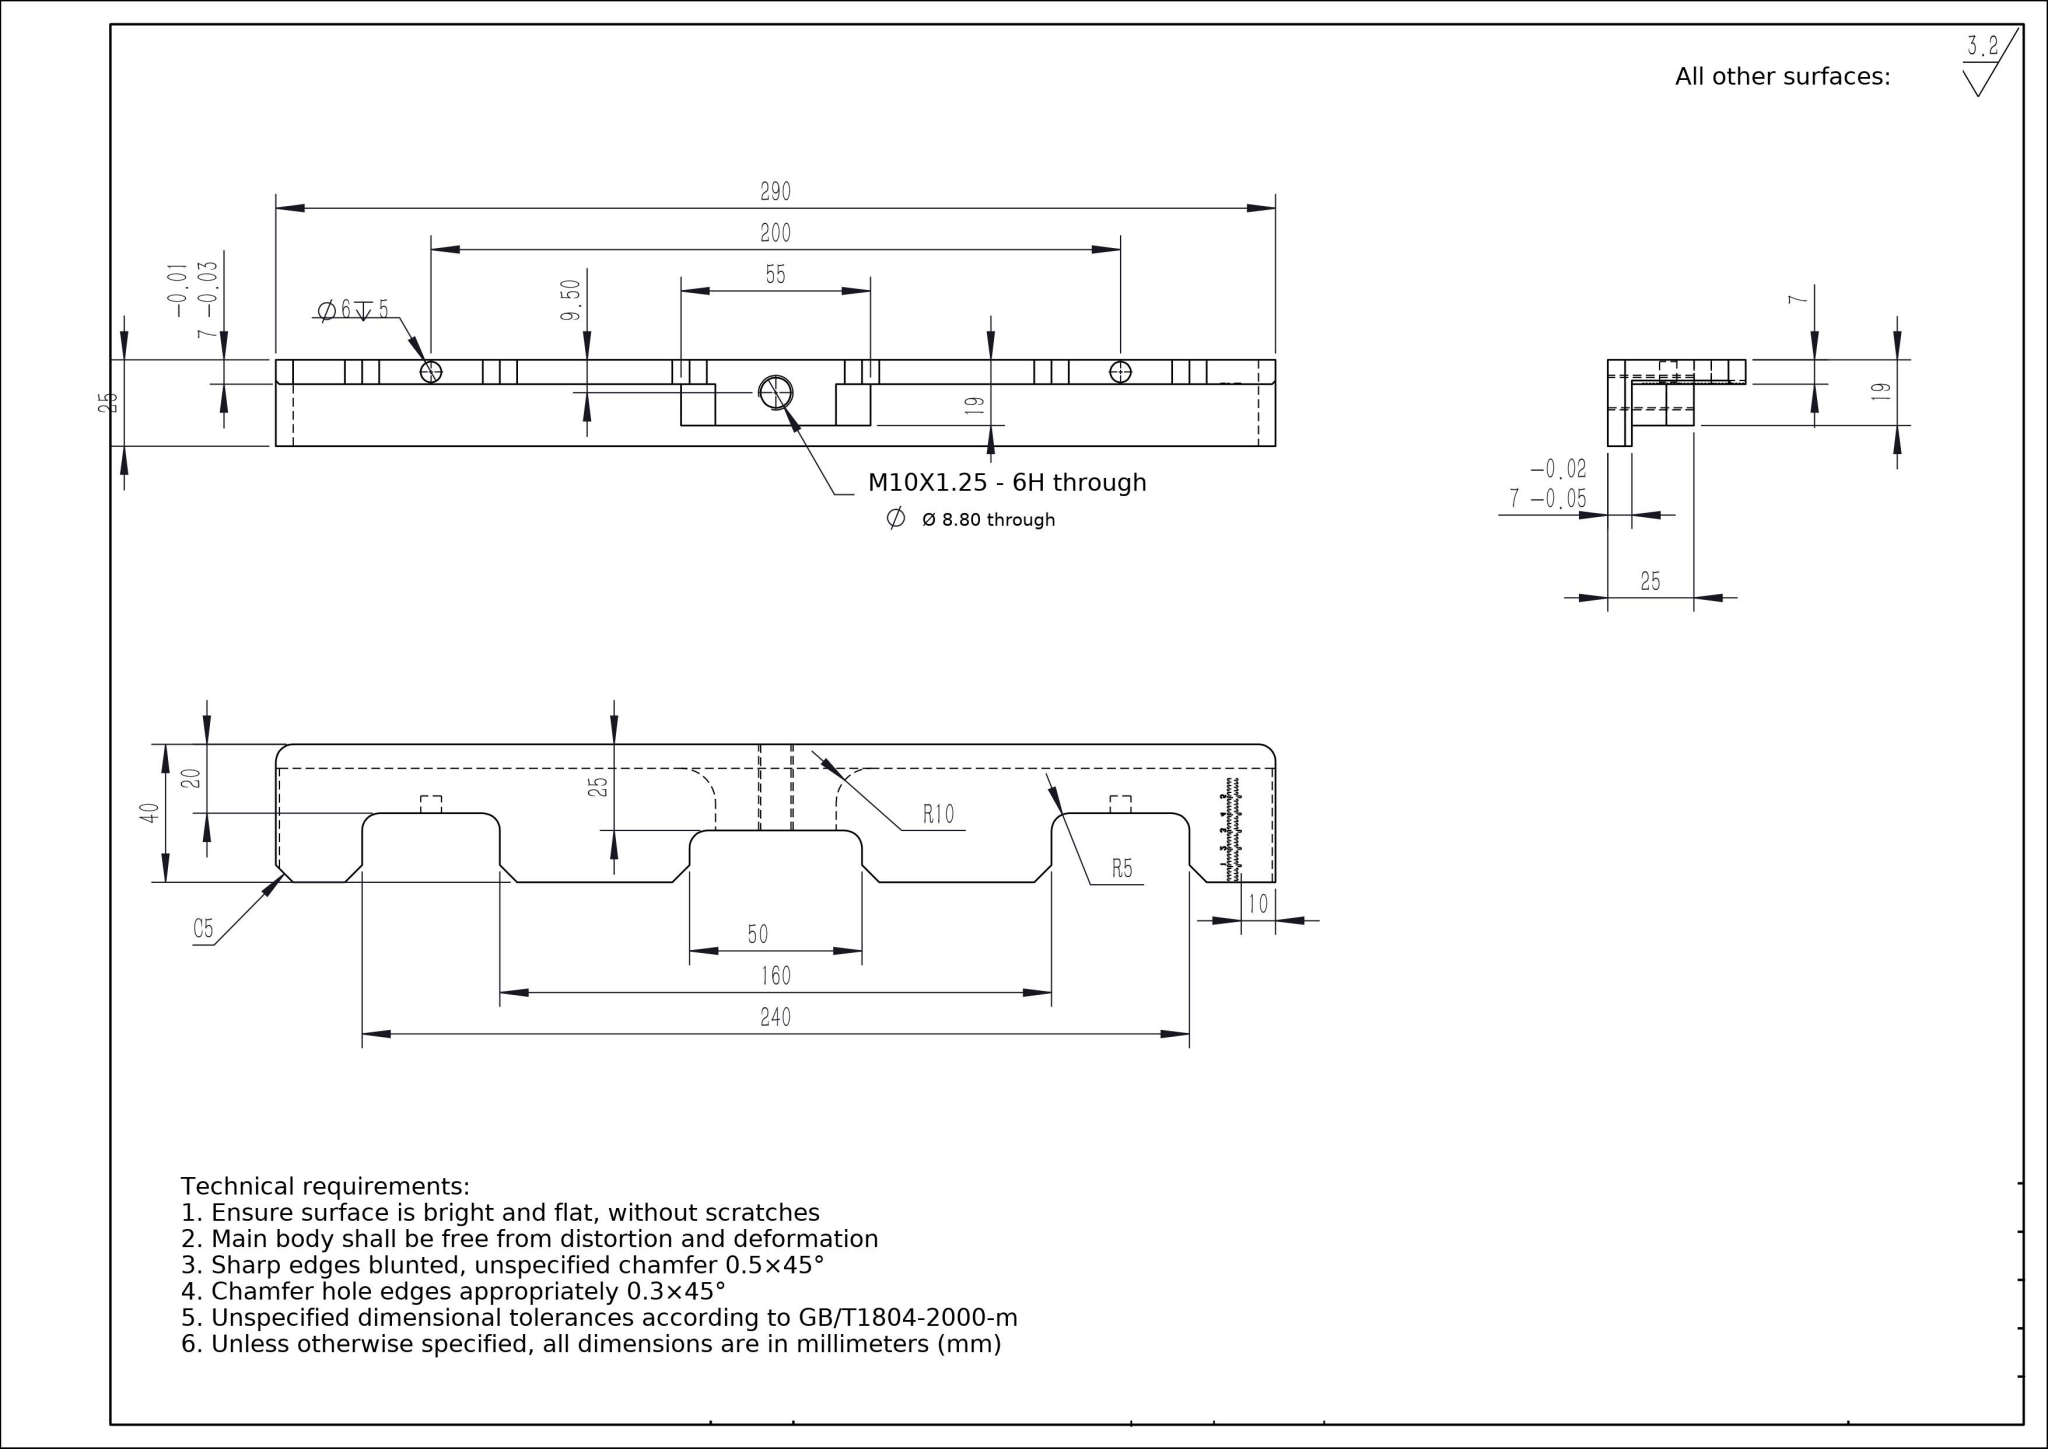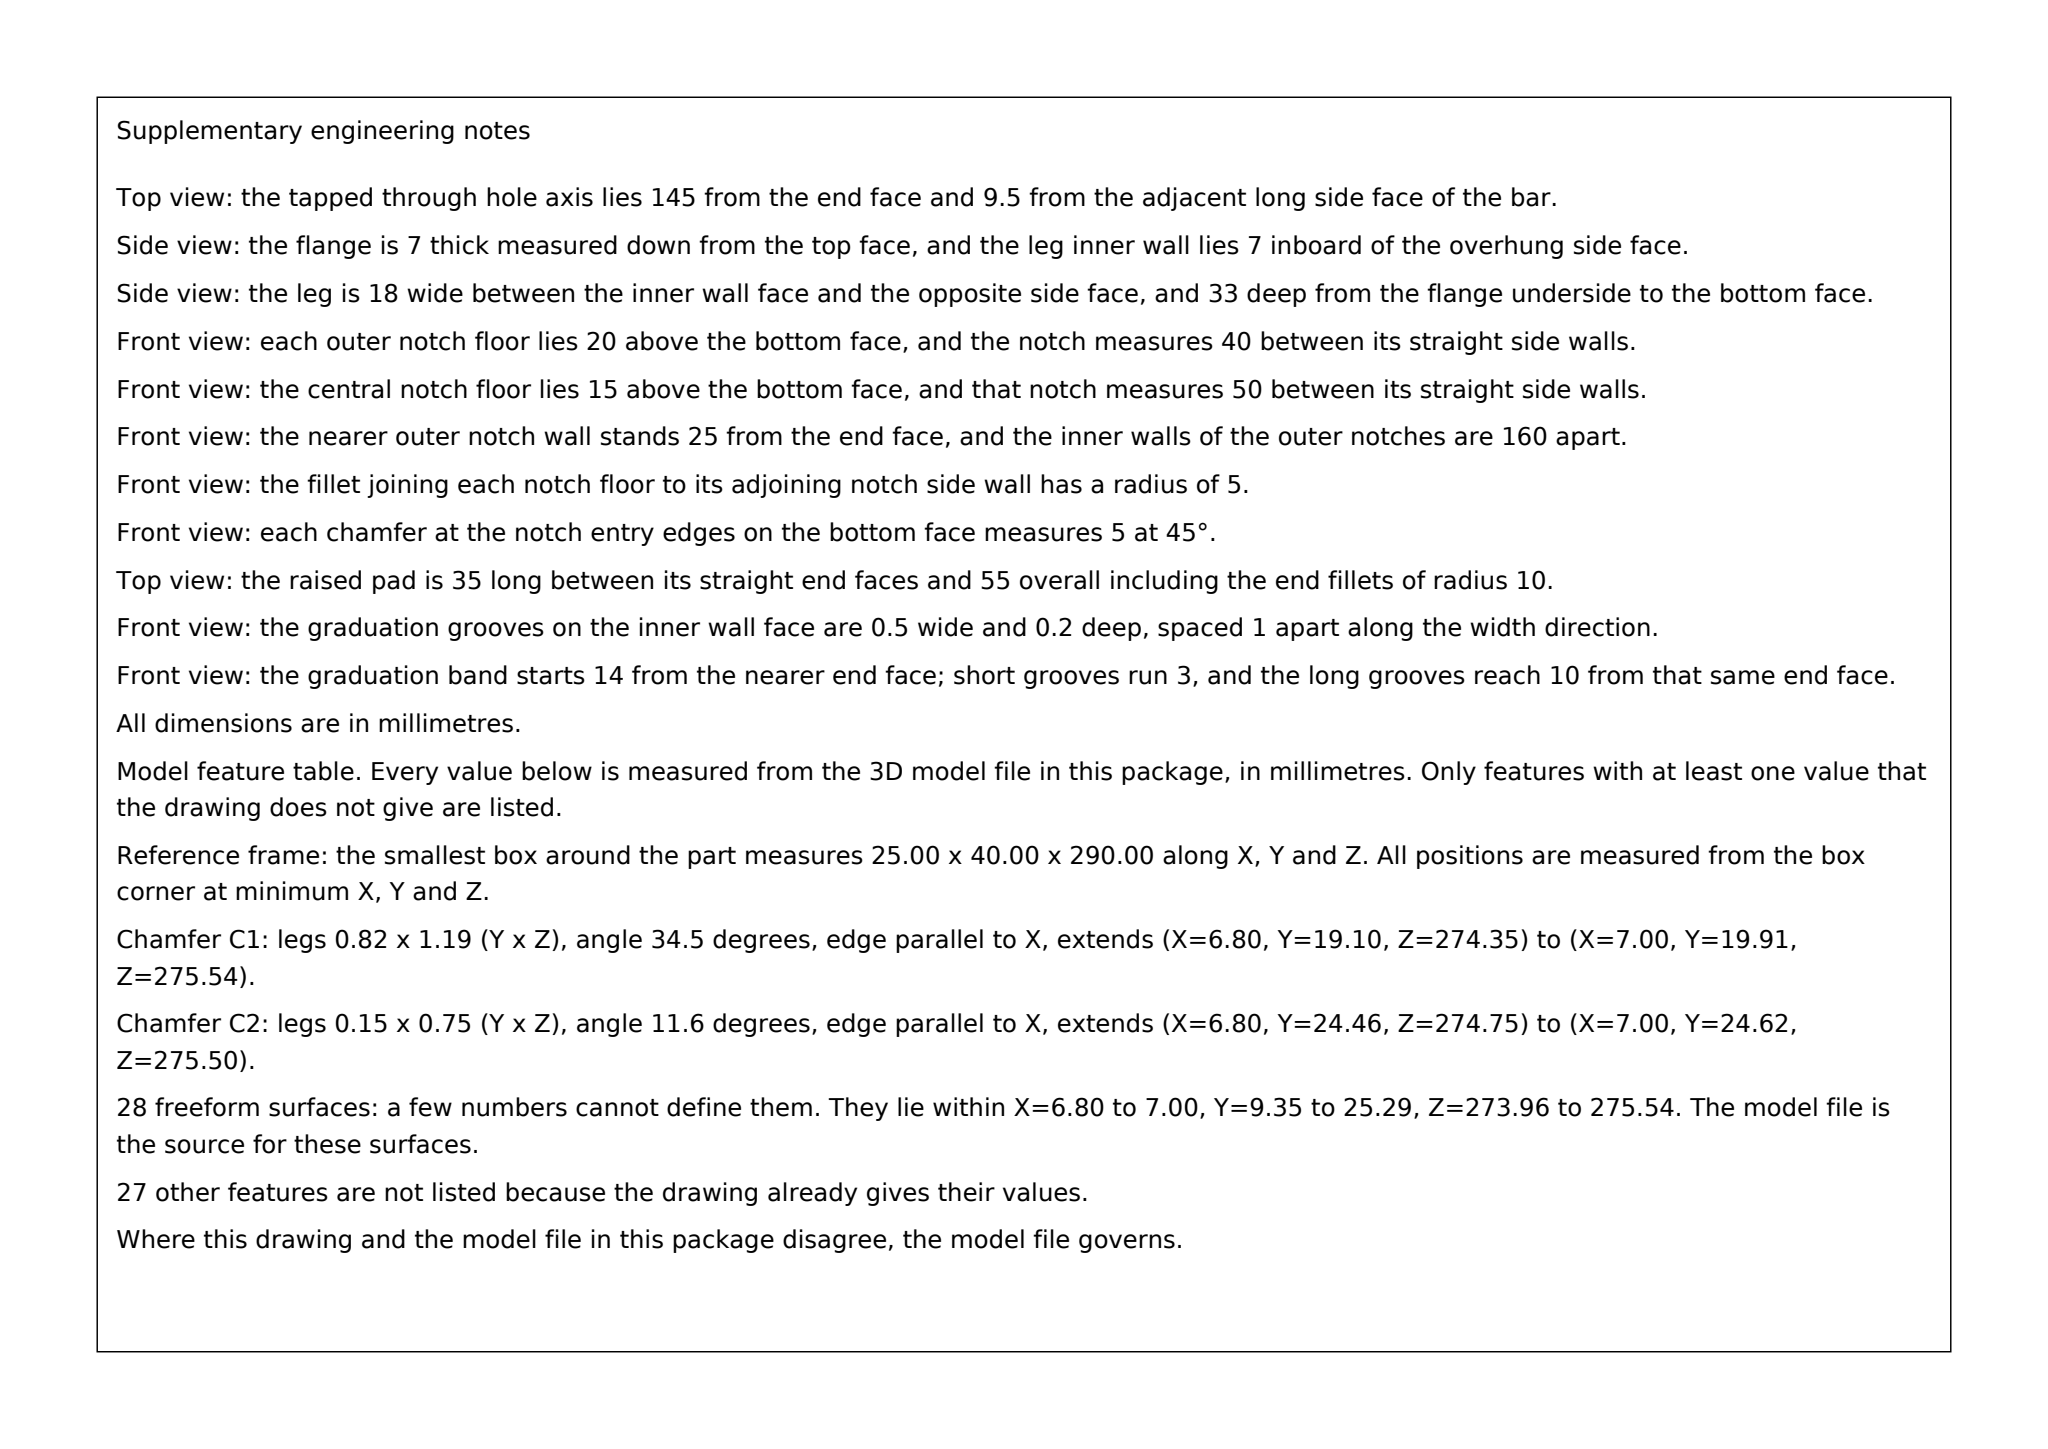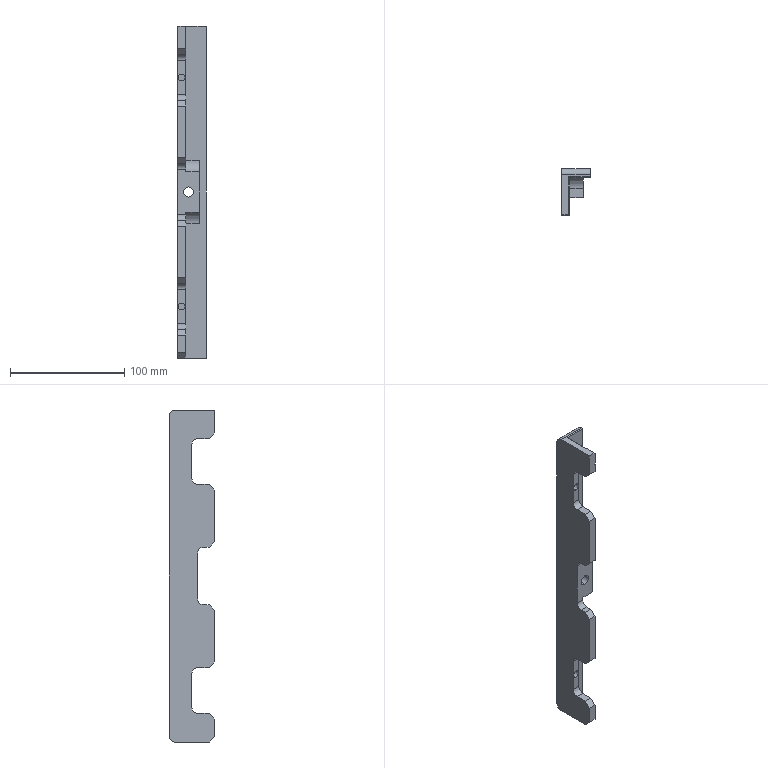Part | SolidWorks | mm | 1 solid | 269 faces | box 25 x 40 x 290 mm | volume 106866 mm3 | plane 225 | spline 28 | cylinder 16 | commonest cylinder face diameters 10 x8 6 x4 8.8 x2 20 x2
Drawing notes:
2X Ø6 DP 5 AT 45 & 245 FROM LH END, 3.5 FROM FRONT FACE | from the solid: cyl dia6 axis y, x=3.5, z=45 & 245, length 5
PADS START AT 25, 120, 225 FROM LH END; WIDTHS 40, 50, 40 | from the solid: z planes 0/25/65/120 + symmetry about z=145 of 290 length: pads 25-65,120-170,225-265
R10 ALL PAD-TO-BASE TRANSITIONS, R5 PAD TOP CORNERS TYP | from the solid: pad transitions at z=25,65,120,170,225,265; R10/R5 callouts in front view
2X Ø10 THRU AT 5 & 285 FROM LH END, 35 UP FROM BTM | from the solid: cyl dia10 axis x, y=35, z=5 & 285, length 25 = full width
4X Ø10 DP 7 AT 30, 60, 230, 260 FROM LH END, 15 UP FROM BTM | from the solid: cyl dia10 axis x, y=15, z=30/60/230/260, length 7
2X Ø10 DP 7 AT 125 & 165 FROM LH END, 10 UP FROM BTM | from the solid: cyl dia10 axis x, y=10, z=125 & 165, length 7
2X Ø20 DP 12 AT 117.5 & 172.5 FROM LH END, 23 UP FROM BTM | from the solid: cyl dia20 axis x, y=23, z=117.5 & 172.5, length 12
GRADUATION MARKS 0.2 DEEP FROM 7 THK FACE | from the solid: Mark floors on plane x=6.8 vs engraved face x=7.0 -> 0.2 deep
GRADUATIONS SPAN 30 UP FROM BOTTOM EDGE, 0.5 PITCH, 61 MARKS | from the solid: Mark planes y=0.0 to y=30.0 every 0.5 (61 planes); bbox Y=40
GRADUATED ZONE 10 WIDE ON 7 THK FACE (SEE SIDE VIEW) | from the solid: Engraved face is x=7.0 plane; 10 wide zone already dimensioned
M10X1.25-6H THRU (Ø8.80 TAP DRILL), AXIS 145 FROM LH END AND 9.5 FROM FRONT FACE, THRU FULL 25 WIDTH | from the solid: cylinder dia 8.80, axis y, pos [x=9.5, z=145.0], length 25.0
GRADUATED FACE IS THE 7 THK FACE (X=7.0); MARK FLOORS AT X=6.8 (0.2 DEEP), 61 MARKS AT 0.5 PITCH FROM Y=0 TO Y=30 | from the solid: axis_planes x=7.0 and x=6.8 (35 faces); y planes at 0.0,0.5,...,30.0
GRADUATION MARKS: 61 MARKS AT 0.5 PITCH, FIRST MARK AT BOTTOM EDGE (0) AND LAST AT 30 UP FROM BTM; MARK FLOOR AT 6.8 FROM BACK FACE (0.2 DEEP FROM 7 THK FACE) | from the solid: axis_planes y = 0.0 through 30.0 in 0.5 increments (61 planes); axis_planes x = 6.8 (35) vs x = 7.0 face
GRADUATIONS ON 7 THK FACE: 61 MARKS AT 0.5 PITCH, FIRST MARK AT BOTTOM EDGE, LAST AT 30 UP; MARKS 0.2 DEEP (FROM FACE AT 7.0 TO 6.8) | from the solid: axis_planes normal y at 0.0 through 30.0 in 0.5 steps (61 marks); axis_planes normal x at 7.0 (face) and 6.8 (mark floor, 35 faces)
build123d program:
from build123d import *

# Parameters (mm, degrees)
SKETCH1_W               = 25
SKETCH1_H               = 40
BOSS_EXTRUDE1_DEPTH     = 290
SKETCH2_W               = 18
SKETCH2_H               = 33
CUT_EXTRUDE1_DEPTH      = 290
FILLET1_R               = 5
SKETCH3_W               = 40
SKETCH3_H               = 20
CUT_EXTRUDE2_DEPTH      = 300
FILLET4_R               = 5
SKETCH4_R               = 3
CUT_EXTRUDE3_DEPTH      = 5
SKETCH5_W               = 50
SKETCH5_H               = 30
CUT_EXTRUDE4_DEPTH      = 20
FILLET5_R               = 5
CHAMFER2_SIZE           = 5
SKETCH6_W               = 35
SKETCH6_H               = 18
BOSS_EXTRUDE2_DEPTH     = 12
FILLET6_R               = 10
M10X1_25_TAPPED_HOLE1_D = 8.8
CHAMFER3_SIZE           = 1
SKETCH11_W              = 3
SKETCH11_H              = 0.5
CUT_EXTRUDE6_DEPTH      = 0.2
SKETCH13_W              = 1
SKETCH13_H              = 0.5
CUT_EXTRUDE7_DEPTH      = 0.2
CUT_EXTRUDE8_DEPTH      = 0.2


with BuildPart() as part:
    # Sketch1 → Boss-Extrude1 (new body)
    with BuildSketch(Plane.XY):
        Rectangle(SKETCH1_W, SKETCH1_H)
    extrude(amount=BOSS_EXTRUDE1_DEPTH)

    # Sketch2 → Cut-Extrude1 (cut)
    with BuildSketch(Plane.XY.offset(290)):
        with Locations((3.5, -3.5)):
            Rectangle(SKETCH2_W, SKETCH2_H)
    extrude(amount=-CUT_EXTRUDE1_DEPTH, mode=Mode.SUBTRACT)

    # Fillet1
    fillet1_edges = [part.edges().sort_by_distance(p)[0] for p in [
        (0, 20, 0),
        (0, 20, 290),
    ]]
    fillet(fillet1_edges, radius=FILLET1_R)

    # Sketch3 → Cut-Extrude2 (cut)
    with BuildSketch(Plane(origin=(-5.5, 0, 0), x_dir=(0, 0, -1), z_dir=(1, 0, 0))):
        with Locations((-245, -10)):
            Rectangle(SKETCH3_W, SKETCH3_H)
        with Locations((-45, -10)):
            Rectangle(SKETCH3_W, SKETCH3_H)
    extrude(amount=-CUT_EXTRUDE2_DEPTH, mode=Mode.SUBTRACT)

    # Fillet4
    fillet4_edges = [part.edges().sort_by_distance(p)[0] for p in [
        (-9, 0, 265),
        (-9, 0, 225),
        (-9, 0, 65),
        (-9, 0, 25),
    ]]
    fillet(fillet4_edges, radius=FILLET4_R)

    # Sketch4 → Cut-Extrude3 (cut)
    with BuildSketch(Plane.XZ):
        with Locations(Location((-9, 245, 0), (0, 0, 270))):
            Circle(SKETCH4_R)
        with Locations(Location((-9, 45, 0), (0, 0, 90))):
            Circle(SKETCH4_R)
    extrude(amount=-CUT_EXTRUDE3_DEPTH, mode=Mode.SUBTRACT)

    # Sketch5 → Cut-Extrude4 (cut)
    with BuildSketch(Plane(origin=(-5.5, 0, 0), x_dir=(0, 0, -1), z_dir=(1, 0, 0))):
        with Locations((-145, -20)):
            Rectangle(SKETCH5_W, SKETCH5_H)
    extrude(amount=-CUT_EXTRUDE4_DEPTH, mode=Mode.SUBTRACT)

    # Fillet5
    fillet5_edges = [part.edges().sort_by_distance(p)[0] for p in [
        (-9, -5, 120),
        (-9, -5, 170),
    ]]
    fillet(fillet5_edges, radius=FILLET5_R)

    # Chamfer2
    chamfer2_edges = [part.edges().sort_by_distance(p)[0] for p in [
        (-9, -20, 120),
        (-9, -20, 170),
        (-9, -20, 0),
        (-9, -20, 265),
        (-9, -20, 225),
        (-9, -20, 25),
        (-9, -20, 65),
    ]]
    chamfer(chamfer2_edges, length=CHAMFER2_SIZE)

    # Sketch6 → Boss-Extrude2 (add)
    with BuildSketch(Plane(origin=(-5.5, 0, 0), x_dir=(0, 0, -1), z_dir=(1, 0, 0))):
        with Locations((-145, 4)):
            Rectangle(SKETCH6_W, SKETCH6_H)
    extrude(amount=BOSS_EXTRUDE2_DEPTH)

    # Fillet6
    fillet6_edges = [part.edges().sort_by_distance(p)[0] for p in [
        (0.5, 13, 162.5),
        (0.5, 13, 127.5),
    ]]
    fillet(fillet6_edges, radius=FILLET6_R)

    # M10x1.25 Tapped Hole1 (through all)
    with Locations(Plane(origin=(0, -5, 0), x_dir=(-1, 0, 0), z_dir=(0, -1, 0))):
        with Locations((3, -145)):
            Hole(M10X1_25_TAPPED_HOLE1_D / 2)

    # Chamfer3
    chamfer3_edges = [part.edges().sort_by_distance(p)[0] for p in [
        (-5.5, -1, 0),
        (-5.5, -3.5, 290),
    ]]
    chamfer(chamfer3_edges, length=CHAMFER3_SIZE)

    # Sketch11 → Cut-Extrude6 (cut)
    with BuildSketch(Plane(origin=(-5.5, 0, 0), x_dir=(0, 0, -1), z_dir=(1, 0, 0))):
        with Locations((-277.5, -18.25)):
            Rectangle(SKETCH11_W, SKETCH11_H)
        with Locations((-277.5, -19.25)):
            Rectangle(SKETCH11_W, SKETCH11_H)
        with Locations((-277.5, -17.25)):
            Rectangle(SKETCH11_W, SKETCH11_H)
        with Locations((-277.5, -16.25)):
            Rectangle(SKETCH11_W, SKETCH11_H)
        with Locations((-277.5, -15.25)):
            Rectangle(SKETCH11_W, SKETCH11_H)
        with Locations((-277.5, -14.25)):
            Rectangle(SKETCH11_W, SKETCH11_H)
        with Locations((-277.5, -13.25)):
            Rectangle(SKETCH11_W, SKETCH11_H)
        with Locations((-277.5, -12.25)):
            Rectangle(SKETCH11_W, SKETCH11_H)
        with Locations((-277.5, -11.25)):
            Rectangle(SKETCH11_W, SKETCH11_H)
        with Locations((-277.5, -10.25)):
            Rectangle(SKETCH11_W, SKETCH11_H)
        with Locations((-277.5, -9.25)):
            Rectangle(SKETCH11_W, SKETCH11_H)
        with Locations((-277.5, -8.25)):
            Rectangle(SKETCH11_W, SKETCH11_H)
        with Locations((-277.5, -7.25)):
            Rectangle(SKETCH11_W, SKETCH11_H)
        with Locations((-277.5, -6.25)):
            Rectangle(SKETCH11_W, SKETCH11_H)
        with Locations((-277.5, -5.25)):
            Rectangle(SKETCH11_W, SKETCH11_H)
        with Locations((-277.5, -4.25)):
            Rectangle(SKETCH11_W, SKETCH11_H)
        with Locations((-277.5, -3.25)):
            Rectangle(SKETCH11_W, SKETCH11_H)
        with Locations((-277.5, -2.25)):
            Rectangle(SKETCH11_W, SKETCH11_H)
        with Locations((-277.5, -1.25)):
            Rectangle(SKETCH11_W, SKETCH11_H)
        with Locations((-277.5, -0.25)):
            Rectangle(SKETCH11_W, SKETCH11_H)
        with Locations((-277.5, 0.75)):
            Rectangle(SKETCH11_W, SKETCH11_H)
        with Locations((-277.5, 1.75)):
            Rectangle(SKETCH11_W, SKETCH11_H)
        with Locations((-277.5, 2.75)):
            Rectangle(SKETCH11_W, SKETCH11_H)
        with Locations((-277.5, 3.75)):
            Rectangle(SKETCH11_W, SKETCH11_H)
        with Locations((-277.5, 4.75)):
            Rectangle(SKETCH11_W, SKETCH11_H)
        with Locations((-277.5, 5.75)):
            Rectangle(SKETCH11_W, SKETCH11_H)
        with Locations((-277.5, 6.75)):
            Rectangle(SKETCH11_W, SKETCH11_H)
        with Locations((-277.5, 7.75)):
            Rectangle(SKETCH11_W, SKETCH11_H)
        with Locations((-277.5, 8.75)):
            Rectangle(SKETCH11_W, SKETCH11_H)
        with Locations((-277.5, 9.75)):
            Rectangle(SKETCH11_W, SKETCH11_H)
    extrude(amount=-CUT_EXTRUDE6_DEPTH, mode=Mode.SUBTRACT)

    # Sketch13 → Cut-Extrude7 (cut)
    with BuildSketch(Plane(origin=(-5.5, 0, 0), x_dir=(0, 0, -1), z_dir=(1, 0, 0))):
        with Locations((-279.5, -15.25)):
            Rectangle(SKETCH13_W, SKETCH13_H)
        with Locations((-279.5, -10.25)):
            Rectangle(SKETCH13_W, SKETCH13_H)
        with Locations((-279.5, -5.25)):
            Rectangle(SKETCH13_W, SKETCH13_H)
        with Locations((-279.5, -0.25)):
            Rectangle(SKETCH13_W, SKETCH13_H)
        with Locations((-279.5, 4.75)):
            Rectangle(SKETCH13_W, SKETCH13_H)
    extrude(amount=-CUT_EXTRUDE7_DEPTH, mode=Mode.SUBTRACT)

    # Sketch14 → Cut-Extrude8 (cut)
    # profile 1 of 5: a face of its own
    with BuildSketch(Plane(origin=(-5.5, 0, 0), x_dir=(0, 0, -1), z_dir=(1, 0, 0))):
        Polygon((-275.5, -15.008), (-275.5, -14.731), (-274, -14.731), (-274, -14.865), (-275.346, -14.865), (-275.346, -15.096), align=None)
    # profile 2 of 5: a face of its own
    with BuildSketch(Plane(origin=(-5.5, 0, 0), x_dir=(0, 0, -1), z_dir=(1, 0, 0))):
        with BuildLine():
            Line((-275.038, -10.519), (-275.038, -10.654))
            add(Edge.make_bspline(
                [(-275.038, -10.654), (-275.056, -10.653), (-275.091, -10.651), (-275.143, -10.643), (-275.191, -10.632), (-275.238, -10.615), (-275.282, -10.595), (-275.323, -10.571), (-275.362, -10.542), (-275.398, -10.509), (-275.431, -10.474), (-275.46, -10.436), (-275.484, -10.395), (-275.504, -10.353), (-275.519, -10.309), (-275.531, -10.263), (-275.537, -10.214), (-275.538, -10.181), (-275.538, -10.165)],
                knots=[0, 0, 0, 0, 1.101, 2.162, 3.184, 4.19, 5.176, 6.163, 7.152, 8.156, 9.156, 10.134, 11.092, 12.041, 13.001, 13.972, 14.969, 16, 16, 16, 16], degree=3))
            add(Edge.make_bspline(
                [(-275.538, -10.165), (-275.538, -10.148), (-275.537, -10.116), (-275.531, -10.069), (-275.521, -10.024), (-275.506, -9.981), (-275.487, -9.941), (-275.464, -9.904), (-275.437, -9.868), (-275.406, -9.836), (-275.373, -9.807), (-275.337, -9.782), (-275.3, -9.76), (-275.261, -9.742), (-275.221, -9.729), (-275.18, -9.719), (-275.137, -9.713), (-275.107, -9.712), (-275.093, -9.712)],
                knots=[0, 0, 0, 0, 1.112, 2.184, 3.213, 4.224, 5.211, 6.196, 7.192, 8.207, 9.22, 10.201, 11.166, 12.121, 13.065, 14.026, 14.997, 16, 16, 16, 16], degree=3))
            add(Edge.make_bspline(
                [(-275.093, -9.712), (-275.072, -9.712), (-275.03, -9.714), (-274.969, -9.726), (-274.91, -9.745), (-274.863, -9.768), (-274.825, -9.792), (-274.793, -9.813), (-274.759, -9.837), (-274.723, -9.866), (-274.684, -9.898), (-274.643, -9.933), (-274.599, -9.973), (-274.57, -10.001), (-274.554, -10.015)],
                knots=[0, 0, 0, 0, 1.184, 2.348, 3.509, 4.696, 5.334, 6.051, 6.844, 7.715, 8.667, 9.695, 10.806, 12, 12, 12, 12], degree=3))
            Line((-274.554, -10.015), (-274.154, -10.39))
            Line((-274.154, -10.39), (-274.154, -9.692))
            Line((-274.154, -9.692), (-274, -9.692))
            Line((-274, -9.692), (-274, -10.712))
            Line((-274, -10.712), (-274.621, -10.13))
            add(Edge.make_bspline(
                [(-274.621, -10.13), (-274.636, -10.116), (-274.664, -10.088), (-274.705, -10.05), (-274.744, -10.015), (-274.779, -9.985), (-274.812, -9.958), (-274.841, -9.935), (-274.868, -9.916), (-274.899, -9.895), (-274.937, -9.875), (-274.984, -9.858), (-275.032, -9.848), (-275.064, -9.847), (-275.081, -9.846)],
                knots=[0, 0, 0, 0, 1.33, 2.554, 3.673, 4.688, 5.603, 6.414, 7.123, 7.735, 8.834, 9.9, 10.944, 12, 12, 12, 12], degree=3))
            add(Edge.make_bspline(
                [(-275.081, -9.846), (-275.091, -9.846), (-275.111, -9.847), (-275.141, -9.852), (-275.169, -9.859), (-275.197, -9.869), (-275.223, -9.883), (-275.248, -9.899), (-275.272, -9.918), (-275.295, -9.94), (-275.316, -9.964), (-275.334, -9.99), (-275.35, -10.017), (-275.363, -10.045), (-275.373, -10.075), (-275.379, -10.106), (-275.384, -10.138), (-275.384, -10.16), (-275.385, -10.172)],
                knots=[0, 0, 0, 0, 0.9914, 1.954, 2.896, 3.839, 4.798, 5.76, 6.748, 7.785, 8.825, 9.84, 10.836, 11.836, 12.849, 13.864, 14.912, 16, 16, 16, 16], degree=3))
            add(Edge.make_bspline(
                [(-275.385, -10.172), (-275.384, -10.183), (-275.384, -10.206), (-275.379, -10.24), (-275.373, -10.273), (-275.362, -10.303), (-275.35, -10.333), (-275.334, -10.36), (-275.316, -10.387), (-275.294, -10.411), (-275.27, -10.434), (-275.244, -10.454), (-275.215, -10.471), (-275.184, -10.486), (-275.151, -10.499), (-275.116, -10.508), (-275.078, -10.515), (-275.052, -10.518), (-275.038, -10.519)],
                knots=[0, 0, 0, 0, 1.031, 2.024, 2.988, 3.934, 4.865, 5.795, 6.73, 7.685, 8.651, 9.612, 10.592, 11.592, 12.625, 13.701, 14.822, 16, 16, 16, 16], degree=3))
        make_face()
    # profile 3 of 5: a face of its own
    with BuildSketch(Plane(origin=(-5.5, 0, 0), x_dir=(0, 0, -1), z_dir=(1, 0, 0))):
        with BuildLine():
            Line((-275.154, -5.327), (-275.154, -5.462))
            add(Edge.make_bspline(
                [(-275.154, -5.462), (-275.169, -5.458), (-275.198, -5.451), (-275.241, -5.436), (-275.281, -5.42), (-275.317, -5.4), (-275.352, -5.379), (-275.384, -5.355), (-275.413, -5.328), (-275.439, -5.299), (-275.463, -5.269), (-275.483, -5.237), (-275.5, -5.203), (-275.514, -5.168), (-275.525, -5.132), (-275.533, -5.094), (-275.538, -5.055), (-275.538, -5.028), (-275.538, -5.015)],
                knots=[0, 0, 0, 0, 1.162, 2.272, 3.344, 4.383, 5.39, 6.38, 7.362, 8.333, 9.296, 10.242, 11.178, 12.116, 13.063, 14.02, 14.995, 16, 16, 16, 16], degree=3))
            add(Edge.make_bspline(
                [(-275.538, -5.015), (-275.538, -4.995), (-275.537, -4.957), (-275.526, -4.9), (-275.509, -4.845), (-275.486, -4.793), (-275.457, -4.744), (-275.423, -4.701), (-275.384, -4.664), (-275.34, -4.633), (-275.294, -4.608), (-275.247, -4.59), (-275.198, -4.579), (-275.165, -4.578), (-275.149, -4.577)],
                knots=[0, 0, 0, 0, 1.083, 2.142, 3.193, 4.256, 5.303, 6.309, 7.297, 8.282, 9.25, 10.18, 11.088, 12, 12, 12, 12], degree=3))
            add(Edge.make_bspline(
                [(-275.149, -4.577), (-275.133, -4.577), (-275.102, -4.578), (-275.057, -4.587), (-275.014, -4.601), (-274.974, -4.62), (-274.936, -4.645), (-274.901, -4.675), (-274.868, -4.711), (-274.85, -4.738), (-274.84, -4.752)],
                knots=[0, 0, 0, 0, 1.025, 2.005, 2.965, 3.921, 4.883, 5.875, 6.906, 8, 8, 8, 8], degree=3))
            add(Edge.make_bspline(
                [(-274.84, -4.752), (-274.832, -4.736), (-274.817, -4.704), (-274.787, -4.662), (-274.753, -4.622), (-274.726, -4.6), (-274.712, -4.59)],
                knots=[0, 0, 0, 0, 1.016, 2.016, 3.001, 4, 4, 4, 4], degree=3))
            add(Edge.make_bspline(
                [(-274.712, -4.59), (-274.702, -4.582), (-274.683, -4.568), (-274.651, -4.55), (-274.619, -4.534), (-274.586, -4.522), (-274.552, -4.512), (-274.518, -4.505), (-274.482, -4.501), (-274.458, -4.5), (-274.446, -4.5)],
                knots=[0, 0, 0, 0, 1.025, 2.033, 3.025, 4.014, 4.992, 5.977, 6.983, 8, 8, 8, 8], degree=3))
            add(Edge.make_bspline(
                [(-274.446, -4.5), (-274.425, -4.501), (-274.383, -4.502), (-274.321, -4.516), (-274.26, -4.537), (-274.202, -4.567), (-274.148, -4.604), (-274.099, -4.648), (-274.058, -4.698), (-274.023, -4.754), (-273.996, -4.815), (-273.976, -4.88), (-273.964, -4.948), (-273.962, -4.995), (-273.962, -5.019)],
                knots=[0, 0, 0, 0, 0.9557, 1.907, 2.875, 3.871, 4.872, 5.854, 6.836, 7.836, 8.849, 9.871, 10.917, 12, 12, 12, 12], degree=3))
            add(Edge.make_bspline(
                [(-273.962, -5.019), (-273.962, -5.035), (-273.963, -5.067), (-273.968, -5.113), (-273.977, -5.157), (-273.989, -5.2), (-274.005, -5.24), (-274.024, -5.278), (-274.047, -5.314), (-274.073, -5.348), (-274.103, -5.38), (-274.137, -5.408), (-274.173, -5.434), (-274.213, -5.457), (-274.256, -5.477), (-274.302, -5.494), (-274.352, -5.509), (-274.386, -5.516), (-274.404, -5.519)],
                knots=[0, 0, 0, 0, 1.049, 2.063, 3.046, 3.999, 4.937, 5.863, 6.793, 7.731, 8.676, 9.628, 10.6, 11.592, 12.626, 13.702, 14.821, 16, 16, 16, 16], degree=3))
            Line((-274.404, -5.519), (-274.404, -5.385))
            add(Edge.make_bspline(
                [(-274.404, -5.385), (-274.392, -5.381), (-274.37, -5.374), (-274.338, -5.363), (-274.308, -5.349), (-274.281, -5.335), (-274.256, -5.32), (-274.234, -5.304), (-274.213, -5.286), (-274.202, -5.273), (-274.197, -5.267)],
                knots=[0, 0, 0, 0, 1.198, 2.331, 3.408, 4.417, 5.372, 6.289, 7.163, 8, 8, 8, 8], degree=3))
            add(Edge.make_bspline(
                [(-274.197, -5.267), (-274.19, -5.259), (-274.177, -5.242), (-274.161, -5.215), (-274.146, -5.186), (-274.135, -5.155), (-274.126, -5.123), (-274.12, -5.089), (-274.116, -5.053), (-274.116, -5.029), (-274.115, -5.017)],
                knots=[0, 0, 0, 0, 0.9461, 1.889, 2.845, 3.81, 4.801, 5.829, 6.891, 8, 8, 8, 8], degree=3))
            add(Edge.make_bspline(
                [(-274.115, -5.017), (-274.116, -5.002), (-274.116, -4.975), (-274.121, -4.935), (-274.128, -4.897), (-274.139, -4.861), (-274.152, -4.827), (-274.168, -4.796), (-274.188, -4.766), (-274.21, -4.739), (-274.234, -4.715), (-274.259, -4.693), (-274.286, -4.675), (-274.313, -4.66), (-274.341, -4.649), (-274.371, -4.641), (-274.402, -4.635), (-274.422, -4.635), (-274.433, -4.635)],
                knots=[0, 0, 0, 0, 1.217, 2.38, 3.494, 4.572, 5.61, 6.639, 7.649, 8.668, 9.67, 10.625, 11.543, 12.441, 13.322, 14.205, 15.095, 16, 16, 16, 16], degree=3))
            add(Edge.make_bspline(
                [(-274.433, -4.635), (-274.447, -4.635), (-274.475, -4.637), (-274.516, -4.647), (-274.555, -4.663), (-274.593, -4.686), (-274.627, -4.714), (-274.658, -4.747), (-274.683, -4.784), (-274.701, -4.819), (-274.713, -4.85), (-274.721, -4.876), (-274.728, -4.906), (-274.734, -4.938), (-274.74, -4.973), (-274.744, -5.012), (-274.748, -5.053), (-274.749, -5.081), (-274.75, -5.096)],
                knots=[0, 0, 0, 0, 1.071, 2.136, 3.216, 4.346, 5.486, 6.622, 7.776, 8.964, 9.598, 10.305, 11.07, 11.915, 12.824, 13.806, 14.869, 16, 16, 16, 16], degree=3))
            Line((-274.75, -5.096), (-274.904, -5.096))
            add(Edge.make_bspline(
                [(-274.904, -5.096), (-274.904, -5.078), (-274.905, -5.041), (-274.912, -4.988), (-274.923, -4.937), (-274.938, -4.89), (-274.957, -4.847), (-274.978, -4.809), (-275.002, -4.778), (-275.029, -4.754), (-275.057, -4.735), (-275.086, -4.721), (-275.117, -4.713), (-275.139, -4.712), (-275.149, -4.712)],
                knots=[0, 0, 0, 0, 1.322, 2.589, 3.817, 5.012, 6.141, 7.155, 8.081, 8.93, 9.728, 10.489, 11.24, 12, 12, 12, 12], degree=3))
            add(Edge.make_bspline(
                [(-275.149, -4.712), (-275.157, -4.712), (-275.173, -4.712), (-275.196, -4.717), (-275.218, -4.723), (-275.239, -4.733), (-275.259, -4.745), (-275.279, -4.759), (-275.297, -4.777), (-275.315, -4.797), (-275.332, -4.819), (-275.346, -4.842), (-275.358, -4.867), (-275.368, -4.894), (-275.375, -4.922), (-275.381, -4.951), (-275.384, -4.982), (-275.384, -5.003), (-275.385, -5.013)],
                knots=[0, 0, 0, 0, 0.8843, 1.759, 2.623, 3.489, 4.373, 5.295, 6.256, 7.274, 8.302, 9.333, 10.377, 11.441, 12.52, 13.637, 14.799, 16, 16, 16, 16], degree=3))
            add(Edge.make_bspline(
                [(-275.385, -5.013), (-275.384, -5.03), (-275.383, -5.064), (-275.373, -5.112), (-275.356, -5.156), (-275.337, -5.191), (-275.318, -5.216), (-275.301, -5.234), (-275.282, -5.252), (-275.261, -5.268), (-275.238, -5.284), (-275.212, -5.299), (-275.184, -5.314), (-275.164, -5.322), (-275.154, -5.327)],
                knots=[0, 0, 0, 0, 1.473, 2.876, 4.222, 5.565, 6.25, 6.953, 7.687, 8.464, 9.284, 10.136, 11.041, 12, 12, 12, 12], degree=3))
        make_face()
    # profile 4 of 5: a face of its own
    with BuildSketch(Plane(origin=(-5.5, 0, 0), x_dir=(0, 0, -1), z_dir=(1, 0, 0))):
        Polygon((-275.538, -0.08504), (-275.538, -0.05769), (-274.5, -0.05769), (-274.5, 0.1154), (-274.346, 0.1154), (-274.346, -0.05769), (-274, -0.05769), (-274, -0.1923), (-274.346, -0.1923), (-274.346, -0.9038), align=None)
        Polygon((-274.5, -0.1923), (-275.151, -0.1923), (-274.5, -0.6394), align=None, mode=Mode.SUBTRACT)
    # profile 5 of 5: a face of its own
    with BuildSketch(Plane(origin=(-5.5, 0, 0), x_dir=(0, 0, -1), z_dir=(1, 0, 0))):
        with BuildLine():
            Line((-275.5, 5.231), (-275.346, 5.231))
            Line((-275.346, 5.231), (-275.346, 4.721))
            Line((-275.346, 4.721), (-274.952, 4.64))
            add(Edge.make_bspline(
                [(-274.952, 4.64), (-274.956, 4.656), (-274.965, 4.686), (-274.974, 4.732), (-274.98, 4.775), (-274.98, 4.803), (-274.981, 4.816)],
                knots=[0, 0, 0, 0, 1.1, 2.132, 3.096, 4, 4, 4, 4], degree=3))
            add(Edge.make_bspline(
                [(-274.981, 4.816), (-274.98, 4.833), (-274.98, 4.866), (-274.973, 4.914), (-274.963, 4.96), (-274.947, 5.004), (-274.928, 5.046), (-274.904, 5.084), (-274.876, 5.121), (-274.844, 5.156), (-274.808, 5.187), (-274.77, 5.214), (-274.729, 5.237), (-274.686, 5.256), (-274.64, 5.271), (-274.592, 5.281), (-274.542, 5.287), (-274.508, 5.288), (-274.49, 5.288)],
                knots=[0, 0, 0, 0, 1.053, 2.07, 3.053, 4.021, 4.973, 5.926, 6.892, 7.882, 8.877, 9.857, 10.831, 11.813, 12.813, 13.837, 14.897, 16, 16, 16, 16], degree=3))
            add(Edge.make_bspline(
                [(-274.49, 5.288), (-274.478, 5.288), (-274.454, 5.288), (-274.418, 5.285), (-274.382, 5.279), (-274.348, 5.272), (-274.314, 5.262), (-274.281, 5.25), (-274.249, 5.236), (-274.218, 5.22), (-274.188, 5.203), (-274.16, 5.183), (-274.133, 5.162), (-274.108, 5.14), (-274.085, 5.116), (-274.064, 5.09), (-274.045, 5.064), (-274.027, 5.035), (-274.012, 5.005), (-273.999, 4.974), (-273.987, 4.942), (-273.978, 4.909), (-273.97, 4.875), (-273.965, 4.839), (-273.962, 4.803), (-273.962, 4.778), (-273.962, 4.765)],
                knots=[0, 0, 0, 0, 1.056, 2.099, 3.123, 4.141, 5.141, 6.151, 7.163, 8.173, 9.178, 10.167, 11.141, 12.097, 13.052, 14.005, 14.954, 15.917, 16.885, 17.854, 18.829, 19.818, 20.826, 21.858, 22.918, 24, 24, 24, 24], degree=3))
            add(Edge.make_bspline(
                [(-273.962, 4.765), (-273.962, 4.75), (-273.962, 4.721), (-273.969, 4.678), (-273.977, 4.636), (-273.99, 4.597), (-274.007, 4.559), (-274.027, 4.523), (-274.052, 4.489), (-274.079, 4.457), (-274.11, 4.427), (-274.142, 4.401), (-274.177, 4.377), (-274.215, 4.357), (-274.254, 4.339), (-274.296, 4.326), (-274.339, 4.315), (-274.369, 4.31), (-274.385, 4.308)],
                knots=[0, 0, 0, 0, 1.047, 2.06, 3.044, 4.012, 4.974, 5.932, 6.91, 7.901, 8.899, 9.877, 10.858, 11.851, 12.847, 13.869, 14.917, 16, 16, 16, 16], degree=3))
            Line((-274.385, 4.308), (-274.385, 4.442))
            add(Edge.make_bspline(
                [(-274.385, 4.442), (-274.37, 4.446), (-274.343, 4.452), (-274.304, 4.466), (-274.27, 4.483), (-274.239, 4.504), (-274.212, 4.527), (-274.189, 4.555), (-274.167, 4.586), (-274.149, 4.621), (-274.134, 4.657), (-274.123, 4.695), (-274.117, 4.734), (-274.116, 4.76), (-274.115, 4.773)],
                knots=[0, 0, 0, 0, 1.136, 2.184, 3.172, 4.1, 5.023, 5.957, 6.928, 7.937, 8.96, 9.976, 10.982, 12, 12, 12, 12], degree=3))
            add(Edge.make_bspline(
                [(-274.115, 4.773), (-274.116, 4.786), (-274.116, 4.811), (-274.122, 4.848), (-274.13, 4.884), (-274.142, 4.919), (-274.157, 4.952), (-274.176, 4.983), (-274.198, 5.014), (-274.224, 5.042), (-274.252, 5.068), (-274.281, 5.091), (-274.313, 5.11), (-274.346, 5.127), (-274.381, 5.139), (-274.418, 5.148), (-274.456, 5.153), (-274.482, 5.153), (-274.496, 5.154)],
                knots=[0, 0, 0, 0, 1.027, 2.023, 3.003, 3.969, 4.933, 5.915, 6.908, 7.936, 8.956, 9.957, 10.943, 11.922, 12.908, 13.905, 14.933, 16, 16, 16, 16], degree=3))
            add(Edge.make_bspline(
                [(-274.496, 5.154), (-274.508, 5.154), (-274.531, 5.153), (-274.566, 5.148), (-274.598, 5.141), (-274.629, 5.13), (-274.659, 5.116), (-274.686, 5.099), (-274.712, 5.079), (-274.735, 5.056), (-274.757, 5.03), (-274.776, 5.002), (-274.791, 4.972), (-274.804, 4.94), (-274.815, 4.906), (-274.822, 4.87), (-274.826, 4.832), (-274.827, 4.806), (-274.827, 4.792)],
                knots=[0, 0, 0, 0, 1.046, 2.038, 3.014, 3.956, 4.89, 5.813, 6.763, 7.723, 8.693, 9.666, 10.64, 11.636, 12.663, 13.729, 14.832, 16, 16, 16, 16], degree=3))
            add(Edge.make_bspline(
                [(-274.827, 4.792), (-274.827, 4.78), (-274.826, 4.756), (-274.822, 4.72), (-274.816, 4.681), (-274.808, 4.64), (-274.797, 4.598), (-274.784, 4.554), (-274.768, 4.508), (-274.756, 4.477), (-274.75, 4.462)],
                knots=[0, 0, 0, 0, 0.8176, 1.688, 2.601, 3.572, 4.59, 5.671, 6.803, 8, 8, 8, 8], degree=3))
            Line((-274.75, 4.462), (-275.5, 4.615))
            Line((-275.5, 4.615), (-275.5, 5.231))
        make_face()
    extrude(amount=-CUT_EXTRUDE8_DEPTH, mode=Mode.SUBTRACT)


solid = part.part